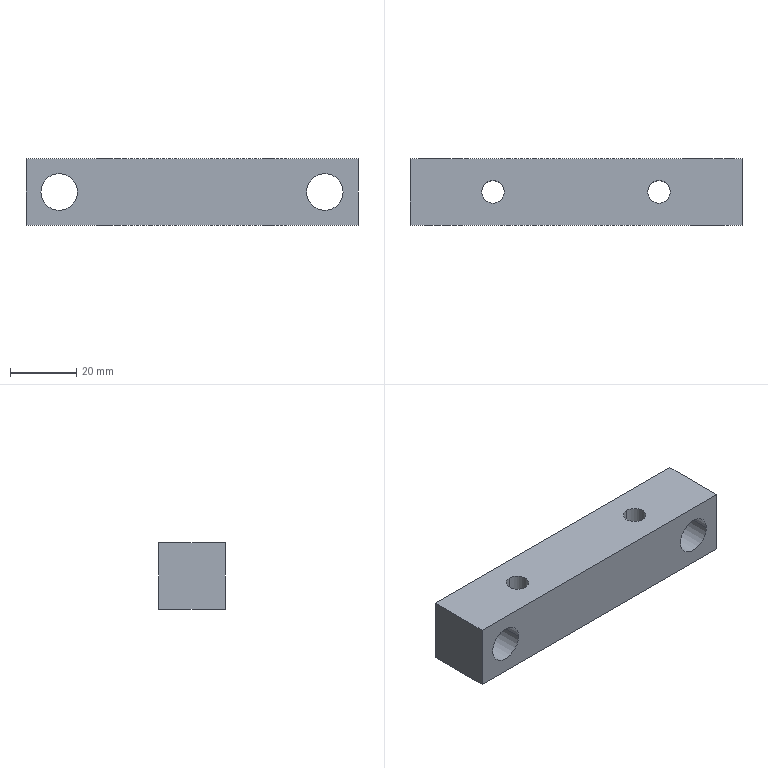Component | SolidWorks | MotorPlateFixingBlock-1 | 1 solid | 20 faces | box 100 x 20 x 20 mm | volume 33112 mm3 | cylinder 12 | plane 8 | commonest cylinder face diameters 6.8 x4 15 x4 11 x4
build123d program:
from build123d import *

# Parameters (mm, degrees)
SKETCH1_W                                        = 100
SKETCH1_H                                        = 20
EXTRUDE1_DEPTH                                   = 20
M10_HEX_SOCKET_HEAD_CAP_SCREW_CBORE1_D           = 11
M10_HEX_SOCKET_HEAD_CAP_SCREW_CBORE1_CBORE_D     = 15
M10_HEX_SOCKET_HEAD_CAP_SCREW_CBORE1_CBORE_DEPTH = 10
M8_TAPPED_HOLE1_D                                = 6.8
M8_TAPPED_HOLE1_DEPTH                            = 22.25
M8_TAPPED_HOLE1_TIP                              = 2.043


with BuildPart() as part:
    # Sketch1 → Extrude1 (new body)
    with BuildSketch(Plane.XY):
        with Locations((27.11, 12.594)):
            Rectangle(SKETCH1_W, SKETCH1_H)
    extrude(amount=EXTRUDE1_DEPTH)

    # M10 Hex Socket Head Cap Screw CBORE1 (through all)
    with Locations(Plane.XY.offset(20)):
        with Locations((67.11, 12.594), (-12.89, 12.594)):
            CounterBoreHole(M10_HEX_SOCKET_HEAD_CAP_SCREW_CBORE1_D / 2, M10_HEX_SOCKET_HEAD_CAP_SCREW_CBORE1_CBORE_D / 2, M10_HEX_SOCKET_HEAD_CAP_SCREW_CBORE1_CBORE_DEPTH)

    # M8 Tapped Hole1
    with Locations(Plane(origin=(0, 22.594, 0), x_dir=(-1, 0, 0), z_dir=(0, 1, 0))):
        with Locations((-52.11, 10), (-2.11, 10)):
            Hole(M8_TAPPED_HOLE1_D / 2, depth=M8_TAPPED_HOLE1_DEPTH)
            with Locations((0, 0, -(M8_TAPPED_HOLE1_DEPTH + M8_TAPPED_HOLE1_TIP / 2))):  # 118° drill point
                Cone(0, M8_TAPPED_HOLE1_D / 2, M8_TAPPED_HOLE1_TIP, mode=Mode.SUBTRACT)


solid = part.part

# Placed as in the assembly
solid = solid.moved(Location((-188.054, 598.983, 240.383), (-90, 0, 0)))
STEP:
#1=CARTESIAN_POINT('',(-7.321,23.842,8.574));
#2=VERTEX_POINT('',#1);
#3=CARTESIAN_POINT('',(-7.321,24.11,8.574));
#4=VERTEX_POINT('',#3);
#5=CARTESIAN_POINT('',(-7.321,23.976,8.574));
#6=DIRECTION('',(0.,0.,1.));
#7=DIRECTION('',(0.,1.,0.));
#8=AXIS2_PLACEMENT_3D('',#5,#6,#7);
#9=CIRCLE('',#8,0.1339);
#10=EDGE_CURVE('',#2,#4,#9,.T.);
#11=ORIENTED_EDGE('',*,*,#10,.F.);
#12=CARTESIAN_POINT('',(-7.321,23.842,9.362));
#13=VERTEX_POINT('',#12);
#14=CARTESIAN_POINT('',(-7.321,23.842,9.362));
#15=DIRECTION('',(0.,0.,1.));
#16=VECTOR('',#15,39.37);
#17=LINE('',#14,#16);
#18=EDGE_CURVE('',#2,#13,#17,.T.);
#19=ORIENTED_EDGE('',*,*,#18,.T.);
#20=CARTESIAN_POINT('',(-7.321,24.11,9.362));
#21=VERTEX_POINT('',#20);
#22=CARTESIAN_POINT('',(-7.321,23.976,9.362));
#23=DIRECTION('',(0.,0.,1.));
#24=DIRECTION('',(0.,1.,0.));
#25=AXIS2_PLACEMENT_3D('',#22,#23,#24);
#26=CIRCLE('',#25,0.1339);
#27=EDGE_CURVE('',#13,#21,#26,.T.);
#28=ORIENTED_EDGE('',*,*,#27,.T.);
#29=CARTESIAN_POINT('',(-7.321,24.11,9.362));
#30=DIRECTION('',(0.,0.,1.));
#31=VECTOR('',#30,39.37);
#32=LINE('',#29,#31);
#33=EDGE_CURVE('',#4,#21,#32,.T.);
#34=ORIENTED_EDGE('',*,*,#33,.F.);
#35=EDGE_LOOP('',(#11,#19,#28,#34));
#36=FACE_OUTER_BOUND('',#35,.T.);
#37=CARTESIAN_POINT('',(-7.321,23.976,9.362));
#38=DIRECTION('',(0.,0.,1.));
#39=DIRECTION('',(0.,1.,0.));
#40=AXIS2_PLACEMENT_3D('',#37,#38,#39);
#41=CYLINDRICAL_SURFACE('',#40,0.1339);
#42=ADVANCED_FACE('',(#36),#41,.F.);
#43=CARTESIAN_POINT('',(-5.352,23.842,8.574));
#44=VERTEX_POINT('',#43);
#45=CARTESIAN_POINT('',(-5.352,24.11,8.574));
#46=VERTEX_POINT('',#45);
#47=CARTESIAN_POINT('',(-5.352,23.976,8.574));
#48=DIRECTION('',(0.,0.,1.));
#49=DIRECTION('',(0.,1.,0.));
#50=AXIS2_PLACEMENT_3D('',#47,#48,#49);
#51=CIRCLE('',#50,0.1339);
#52=EDGE_CURVE('',#44,#46,#51,.T.);
#53=ORIENTED_EDGE('',*,*,#52,.F.);
#54=CARTESIAN_POINT('',(-5.352,23.842,9.362));
#55=VERTEX_POINT('',#54);
#56=CARTESIAN_POINT('',(-5.352,23.842,9.362));
#57=DIRECTION('',(0.,0.,1.));
#58=VECTOR('',#57,39.37);
#59=LINE('',#56,#58);
#60=EDGE_CURVE('',#44,#55,#59,.T.);
#61=ORIENTED_EDGE('',*,*,#60,.T.);
#62=CARTESIAN_POINT('',(-5.352,24.11,9.362));
#63=VERTEX_POINT('',#62);
#64=CARTESIAN_POINT('',(-5.352,23.976,9.362));
#65=DIRECTION('',(0.,0.,1.));
#66=DIRECTION('',(0.,1.,0.));
#67=AXIS2_PLACEMENT_3D('',#64,#65,#66);
#68=CIRCLE('',#67,0.1339);
#69=EDGE_CURVE('',#55,#63,#68,.T.);
#70=ORIENTED_EDGE('',*,*,#69,.T.);
#71=CARTESIAN_POINT('',(-5.352,24.11,9.362));
#72=DIRECTION('',(0.,0.,1.));
#73=VECTOR('',#72,39.37);
#74=LINE('',#71,#73);
#75=EDGE_CURVE('',#46,#63,#74,.T.);
#76=ORIENTED_EDGE('',*,*,#75,.F.);
#77=EDGE_LOOP('',(#53,#61,#70,#76));
#78=FACE_OUTER_BOUND('',#77,.T.);
#79=CARTESIAN_POINT('',(-5.352,23.976,9.362));
#80=DIRECTION('',(0.,0.,1.));
#81=DIRECTION('',(0.,1.,0.));
#82=AXIS2_PLACEMENT_3D('',#79,#80,#81);
#83=CYLINDRICAL_SURFACE('',#82,0.1339);
#84=ADVANCED_FACE('',(#78),#83,.F.);
#85=CARTESIAN_POINT('',(-4.466,23.976,8.968));
#86=VERTEX_POINT('',#85);
#87=CARTESIAN_POINT('',(-5.057,23.976,8.968));
#88=VERTEX_POINT('',#87);
#89=CARTESIAN_POINT('',(-4.762,23.976,8.968));
#90=DIRECTION('',(0.,1.,-0.));
#91=DIRECTION('',(-1.,0.,0.));
#92=AXIS2_PLACEMENT_3D('',#89,#90,#91);
#93=CIRCLE('',#92,0.2953);
#94=EDGE_CURVE('',#86,#88,#93,.T.);
#95=ORIENTED_EDGE('',*,*,#94,.F.);
#96=CARTESIAN_POINT('',(-4.466,24.369,8.968));
#97=VERTEX_POINT('',#96);
#98=CARTESIAN_POINT('',(-4.466,24.369,8.968));
#99=DIRECTION('',(0.,1.,-0.));
#100=VECTOR('',#99,39.37);
#101=LINE('',#98,#100);
#102=EDGE_CURVE('',#86,#97,#101,.T.);
#103=ORIENTED_EDGE('',*,*,#102,.T.);
#104=CARTESIAN_POINT('',(-5.057,24.369,8.968));
#105=VERTEX_POINT('',#104);
#106=CARTESIAN_POINT('',(-4.762,24.369,8.968));
#107=DIRECTION('',(0.,1.,-0.));
#108=DIRECTION('',(-1.,0.,0.));
#109=AXIS2_PLACEMENT_3D('',#106,#107,#108);
#110=CIRCLE('',#109,0.2953);
#111=EDGE_CURVE('',#97,#105,#110,.T.);
#112=ORIENTED_EDGE('',*,*,#111,.T.);
#113=CARTESIAN_POINT('',(-5.057,24.369,8.968));
#114=DIRECTION('',(0.,1.,-0.));
#115=VECTOR('',#114,39.37);
#116=LINE('',#113,#115);
#117=EDGE_CURVE('',#88,#105,#116,.T.);
#118=ORIENTED_EDGE('',*,*,#117,.F.);
#119=EDGE_LOOP('',(#95,#103,#112,#118));
#120=FACE_OUTER_BOUND('',#119,.T.);
#121=CARTESIAN_POINT('',(-4.762,24.369,8.968));
#122=DIRECTION('',(0.,1.,-0.));
#123=DIRECTION('',(-1.,0.,0.));
#124=AXIS2_PLACEMENT_3D('',#121,#122,#123);
#125=CYLINDRICAL_SURFACE('',#124,0.2953);
#126=ADVANCED_FACE('',(#120),#125,.F.);
#127=CARTESIAN_POINT('',(-4.545,23.582,8.968));
#128=VERTEX_POINT('',#127);
#129=CARTESIAN_POINT('',(-4.978,23.582,8.968));
#130=VERTEX_POINT('',#129);
#131=CARTESIAN_POINT('',(-4.762,23.582,8.968));
#132=DIRECTION('',(0.,1.,-0.));
#133=DIRECTION('',(-1.,0.,0.));
#134=AXIS2_PLACEMENT_3D('',#131,#132,#133);
#135=CIRCLE('',#134,0.2165);
#136=EDGE_CURVE('',#128,#130,#135,.T.);
#137=ORIENTED_EDGE('',*,*,#136,.F.);
#138=CARTESIAN_POINT('',(-4.545,23.976,8.968));
#139=VERTEX_POINT('',#138);
#140=CARTESIAN_POINT('',(-4.545,24.369,8.968));
#141=DIRECTION('',(0.,1.,-0.));
#142=VECTOR('',#141,39.37);
#143=LINE('',#140,#142);
#144=EDGE_CURVE('',#128,#139,#143,.T.);
#145=ORIENTED_EDGE('',*,*,#144,.T.);
#146=CARTESIAN_POINT('',(-4.978,23.976,8.968));
#147=VERTEX_POINT('',#146);
#148=CARTESIAN_POINT('',(-4.762,23.976,8.968));
#149=DIRECTION('',(0.,1.,-0.));
#150=DIRECTION('',(-1.,0.,0.));
#151=AXIS2_PLACEMENT_3D('',#148,#149,#150);
#152=CIRCLE('',#151,0.2165);
#153=EDGE_CURVE('',#139,#147,#152,.T.);
#154=ORIENTED_EDGE('',*,*,#153,.T.);
#155=CARTESIAN_POINT('',(-4.978,24.369,8.968));
#156=DIRECTION('',(0.,1.,-0.));
#157=VECTOR('',#156,39.37);
#158=LINE('',#155,#157);
#159=EDGE_CURVE('',#130,#147,#158,.T.);
#160=ORIENTED_EDGE('',*,*,#159,.F.);
#161=EDGE_LOOP('',(#137,#145,#154,#160));
#162=FACE_OUTER_BOUND('',#161,.T.);
#163=CARTESIAN_POINT('',(-4.762,24.369,8.968));
#164=DIRECTION('',(0.,1.,-0.));
#165=DIRECTION('',(-1.,0.,0.));
#166=AXIS2_PLACEMENT_3D('',#163,#164,#165);
#167=CYLINDRICAL_SURFACE('',#166,0.2165);
#168=ADVANCED_FACE('',(#162),#167,.F.);
#169=CARTESIAN_POINT('',(-7.616,23.976,8.968));
#170=VERTEX_POINT('',#169);
#171=CARTESIAN_POINT('',(-8.206,23.976,8.968));
#172=VERTEX_POINT('',#171);
#173=CARTESIAN_POINT('',(-7.911,23.976,8.968));
#174=DIRECTION('',(0.,1.,-0.));
#175=DIRECTION('',(-1.,0.,0.));
#176=AXIS2_PLACEMENT_3D('',#173,#174,#175);
#177=CIRCLE('',#176,0.2953);
#178=EDGE_CURVE('',#170,#172,#177,.T.);
#179=ORIENTED_EDGE('',*,*,#178,.F.);
#180=CARTESIAN_POINT('',(-7.616,24.369,8.968));
#181=VERTEX_POINT('',#180);
#182=CARTESIAN_POINT('',(-7.616,24.369,8.968));
#183=DIRECTION('',(0.,1.,-0.));
#184=VECTOR('',#183,39.37);
#185=LINE('',#182,#184);
#186=EDGE_CURVE('',#170,#181,#185,.T.);
#187=ORIENTED_EDGE('',*,*,#186,.T.);
#188=CARTESIAN_POINT('',(-8.206,24.369,8.968));
#189=VERTEX_POINT('',#188);
#190=CARTESIAN_POINT('',(-7.911,24.369,8.968));
#191=DIRECTION('',(0.,1.,-0.));
#192=DIRECTION('',(-1.,0.,0.));
#193=AXIS2_PLACEMENT_3D('',#190,#191,#192);
#194=CIRCLE('',#193,0.2953);
#195=EDGE_CURVE('',#181,#189,#194,.T.);
#196=ORIENTED_EDGE('',*,*,#195,.T.);
#197=CARTESIAN_POINT('',(-8.206,24.369,8.968));
#198=DIRECTION('',(0.,1.,-0.));
#199=VECTOR('',#198,39.37);
#200=LINE('',#197,#199);
#201=EDGE_CURVE('',#172,#189,#200,.T.);
#202=ORIENTED_EDGE('',*,*,#201,.F.);
#203=EDGE_LOOP('',(#179,#187,#196,#202));
#204=FACE_OUTER_BOUND('',#203,.T.);
#205=CARTESIAN_POINT('',(-7.911,24.369,8.968));
#206=DIRECTION('',(0.,1.,-0.));
#207=DIRECTION('',(-1.,0.,0.));
#208=AXIS2_PLACEMENT_3D('',#205,#206,#207);
#209=CYLINDRICAL_SURFACE('',#208,0.2953);
#210=ADVANCED_FACE('',(#204),#209,.F.);
#211=CARTESIAN_POINT('',(-7.695,23.582,8.968));
#212=VERTEX_POINT('',#211);
#213=CARTESIAN_POINT('',(-8.128,23.582,8.968));
#214=VERTEX_POINT('',#213);
#215=CARTESIAN_POINT('',(-7.911,23.582,8.968));
#216=DIRECTION('',(0.,1.,-0.));
#217=DIRECTION('',(-1.,0.,0.));
#218=AXIS2_PLACEMENT_3D('',#215,#216,#217);
#219=CIRCLE('',#218,0.2165);
#220=EDGE_CURVE('',#212,#214,#219,.T.);
#221=ORIENTED_EDGE('',*,*,#220,.F.);
#222=CARTESIAN_POINT('',(-7.695,23.976,8.968));
#223=VERTEX_POINT('',#222);
#224=CARTESIAN_POINT('',(-7.695,24.369,8.968));
#225=DIRECTION('',(0.,1.,-0.));
#226=VECTOR('',#225,39.37);
#227=LINE('',#224,#226);
#228=EDGE_CURVE('',#212,#223,#227,.T.);
#229=ORIENTED_EDGE('',*,*,#228,.T.);
#230=CARTESIAN_POINT('',(-8.128,23.976,8.968));
#231=VERTEX_POINT('',#230);
#232=CARTESIAN_POINT('',(-7.911,23.976,8.968));
#233=DIRECTION('',(0.,1.,-0.));
#234=DIRECTION('',(-1.,0.,0.));
#235=AXIS2_PLACEMENT_3D('',#232,#233,#234);
#236=CIRCLE('',#235,0.2165);
#237=EDGE_CURVE('',#223,#231,#236,.T.);
#238=ORIENTED_EDGE('',*,*,#237,.T.);
#239=CARTESIAN_POINT('',(-8.128,24.369,8.968));
#240=DIRECTION('',(0.,1.,-0.));
#241=VECTOR('',#240,39.37);
#242=LINE('',#239,#241);
#243=EDGE_CURVE('',#214,#231,#242,.T.);
#244=ORIENTED_EDGE('',*,*,#243,.F.);
#245=EDGE_LOOP('',(#221,#229,#238,#244));
#246=FACE_OUTER_BOUND('',#245,.T.);
#247=CARTESIAN_POINT('',(-7.911,24.369,8.968));
#248=DIRECTION('',(0.,1.,-0.));
#249=DIRECTION('',(-1.,0.,0.));
#250=AXIS2_PLACEMENT_3D('',#247,#248,#249);
#251=CYLINDRICAL_SURFACE('',#250,0.2165);
#252=ADVANCED_FACE('',(#246),#251,.F.);
#253=CARTESIAN_POINT('',(-4.368,23.582,9.362));
#254=VERTEX_POINT('',#253);
#255=CARTESIAN_POINT('',(-4.368,23.582,8.574));
#256=VERTEX_POINT('',#255);
#257=CARTESIAN_POINT('',(-4.368,23.582,9.362));
#258=DIRECTION('',(-0.,0.,-1.));
#259=VECTOR('',#258,39.37);
#260=LINE('',#257,#259);
#261=EDGE_CURVE('',#254,#256,#260,.T.);
#262=ORIENTED_EDGE('',*,*,#261,.T.);
#263=CARTESIAN_POINT('',(-4.368,24.369,8.574));
#264=VERTEX_POINT('',#263);
#265=CARTESIAN_POINT('',(-4.368,24.369,8.574));
#266=DIRECTION('',(0.,-1.,0.));
#267=VECTOR('',#266,39.37);
#268=LINE('',#265,#267);
#269=EDGE_CURVE('',#264,#256,#268,.T.);
#270=ORIENTED_EDGE('',*,*,#269,.F.);
#271=CARTESIAN_POINT('',(-4.368,24.369,9.362));
#272=VERTEX_POINT('',#271);
#273=CARTESIAN_POINT('',(-4.368,24.369,9.362));
#274=DIRECTION('',(-0.,0.,-1.));
#275=VECTOR('',#274,39.37);
#276=LINE('',#273,#275);
#277=EDGE_CURVE('',#272,#264,#276,.T.);
#278=ORIENTED_EDGE('',*,*,#277,.F.);
#279=CARTESIAN_POINT('',(-4.368,24.369,9.362));
#280=DIRECTION('',(0.,-1.,0.));
#281=VECTOR('',#280,39.37);
#282=LINE('',#279,#281);
#283=EDGE_CURVE('',#272,#254,#282,.T.);
#284=ORIENTED_EDGE('',*,*,#283,.T.);
#285=EDGE_LOOP('',(#262,#270,#278,#284));
#286=FACE_OUTER_BOUND('',#285,.T.);
#287=CARTESIAN_POINT('',(-4.368,24.369,9.362));
#288=DIRECTION('',(-1.,0.,0.));
#289=DIRECTION('',(0.,0.,1.));
#290=AXIS2_PLACEMENT_3D('',#287,#288,#289);
#291=PLANE('',#290);
#292=ADVANCED_FACE('',(#286),#291,.F.);
#293=CARTESIAN_POINT('',(-7.321,23.976,8.574));
#294=DIRECTION('',(0.,0.,1.));
#295=DIRECTION('',(0.,1.,0.));
#296=AXIS2_PLACEMENT_3D('',#293,#294,#295);
#297=CIRCLE('',#296,0.1339);
#298=EDGE_CURVE('',#4,#2,#297,.T.);
#299=ORIENTED_EDGE('',*,*,#298,.T.);
#300=ORIENTED_EDGE('',*,*,#10,.T.);
#301=EDGE_LOOP('',(#299,#300));
#302=FACE_BOUND('',#301,.T.);
#303=CARTESIAN_POINT('',(-5.352,23.976,8.574));
#304=DIRECTION('',(0.,0.,1.));
#305=DIRECTION('',(0.,1.,0.));
#306=AXIS2_PLACEMENT_3D('',#303,#304,#305);
#307=CIRCLE('',#306,0.1339);
#308=EDGE_CURVE('',#46,#44,#307,.T.);
#309=ORIENTED_EDGE('',*,*,#308,.T.);
#310=ORIENTED_EDGE('',*,*,#52,.T.);
#311=EDGE_LOOP('',(#309,#310));
#312=FACE_BOUND('',#311,.T.);
#313=CARTESIAN_POINT('',(-8.305,23.582,8.574));
#314=VERTEX_POINT('',#313);
#315=CARTESIAN_POINT('',(-4.368,23.582,8.574));
#316=DIRECTION('',(-1.,0.,0.));
#317=VECTOR('',#316,39.37);
#318=LINE('',#315,#317);
#319=EDGE_CURVE('',#256,#314,#318,.T.);
#320=ORIENTED_EDGE('',*,*,#319,.T.);
#321=CARTESIAN_POINT('',(-8.305,24.369,8.574));
#322=VERTEX_POINT('',#321);
#323=CARTESIAN_POINT('',(-8.305,24.369,8.574));
#324=DIRECTION('',(0.,-1.,0.));
#325=VECTOR('',#324,39.37);
#326=LINE('',#323,#325);
#327=EDGE_CURVE('',#322,#314,#326,.T.);
#328=ORIENTED_EDGE('',*,*,#327,.F.);
#329=CARTESIAN_POINT('',(-4.368,24.369,8.574));
#330=DIRECTION('',(-1.,0.,0.));
#331=VECTOR('',#330,39.37);
#332=LINE('',#329,#331);
#333=EDGE_CURVE('',#264,#322,#332,.T.);
#334=ORIENTED_EDGE('',*,*,#333,.F.);
#335=ORIENTED_EDGE('',*,*,#269,.T.);
#336=EDGE_LOOP('',(#320,#328,#334,#335));
#337=FACE_OUTER_BOUND('',#336,.T.);
#338=CARTESIAN_POINT('',(-4.368,24.369,8.574));
#339=DIRECTION('',(0.,0.,1.));
#340=DIRECTION('',(0.,1.,-0.));
#341=AXIS2_PLACEMENT_3D('',#338,#339,#340);
#342=PLANE('',#341);
#343=ADVANCED_FACE('',(#302,#312,#337),#342,.F.);
#344=CARTESIAN_POINT('',(-8.305,23.582,9.362));
#345=VERTEX_POINT('',#344);
#346=CARTESIAN_POINT('',(-8.305,23.582,9.362));
#347=DIRECTION('',(0.,0.,1.));
#348=VECTOR('',#347,39.37);
#349=LINE('',#346,#348);
#350=EDGE_CURVE('',#314,#345,#349,.T.);
#351=ORIENTED_EDGE('',*,*,#350,.T.);
#352=CARTESIAN_POINT('',(-8.305,24.369,9.362));
#353=VERTEX_POINT('',#352);
#354=CARTESIAN_POINT('',(-8.305,24.369,9.362));
#355=DIRECTION('',(0.,-1.,0.));
#356=VECTOR('',#355,39.37);
#357=LINE('',#354,#356);
#358=EDGE_CURVE('',#353,#345,#357,.T.);
#359=ORIENTED_EDGE('',*,*,#358,.F.);
#360=CARTESIAN_POINT('',(-8.305,24.369,9.362));
#361=DIRECTION('',(0.,0.,1.));
#362=VECTOR('',#361,39.37);
#363=LINE('',#360,#362);
#364=EDGE_CURVE('',#322,#353,#363,.T.);
#365=ORIENTED_EDGE('',*,*,#364,.F.);
#366=ORIENTED_EDGE('',*,*,#327,.T.);
#367=EDGE_LOOP('',(#351,#359,#365,#366));
#368=FACE_OUTER_BOUND('',#367,.T.);
#369=CARTESIAN_POINT('',(-8.305,24.369,9.362));
#370=DIRECTION('',(1.,0.,0.));
#371=DIRECTION('',(0.,1.,-0.));
#372=AXIS2_PLACEMENT_3D('',#369,#370,#371);
#373=PLANE('',#372);
#374=ADVANCED_FACE('',(#368),#373,.F.);
#375=CARTESIAN_POINT('',(-7.321,23.976,9.362));
#376=DIRECTION('',(0.,0.,1.));
#377=DIRECTION('',(0.,1.,0.));
#378=AXIS2_PLACEMENT_3D('',#375,#376,#377);
#379=CIRCLE('',#378,0.1339);
#380=EDGE_CURVE('',#21,#13,#379,.T.);
#381=ORIENTED_EDGE('',*,*,#380,.F.);
#382=ORIENTED_EDGE('',*,*,#27,.F.);
#383=EDGE_LOOP('',(#381,#382));
#384=FACE_BOUND('',#383,.T.);
#385=CARTESIAN_POINT('',(-5.352,23.976,9.362));
#386=DIRECTION('',(0.,0.,1.));
#387=DIRECTION('',(0.,1.,0.));
#388=AXIS2_PLACEMENT_3D('',#385,#386,#387);
#389=CIRCLE('',#388,0.1339);
#390=EDGE_CURVE('',#63,#55,#389,.T.);
#391=ORIENTED_EDGE('',*,*,#390,.F.);
#392=ORIENTED_EDGE('',*,*,#69,.F.);
#393=EDGE_LOOP('',(#391,#392));
#394=FACE_BOUND('',#393,.T.);
#395=CARTESIAN_POINT('',(-4.368,23.582,9.362));
#396=DIRECTION('',(1.,0.,0.));
#397=VECTOR('',#396,39.37);
#398=LINE('',#395,#397);
#399=EDGE_CURVE('',#345,#254,#398,.T.);
#400=ORIENTED_EDGE('',*,*,#399,.T.);
#401=ORIENTED_EDGE('',*,*,#283,.F.);
#402=CARTESIAN_POINT('',(-4.368,24.369,9.362));
#403=DIRECTION('',(1.,0.,0.));
#404=VECTOR('',#403,39.37);
#405=LINE('',#402,#404);
#406=EDGE_CURVE('',#353,#272,#405,.T.);
#407=ORIENTED_EDGE('',*,*,#406,.F.);
#408=ORIENTED_EDGE('',*,*,#358,.T.);
#409=EDGE_LOOP('',(#400,#401,#407,#408));
#410=FACE_OUTER_BOUND('',#409,.T.);
#411=CARTESIAN_POINT('',(-4.368,24.369,9.362));
#412=DIRECTION('',(0.,-0.,-1.));
#413=DIRECTION('',(0.,-1.,0.));
#414=AXIS2_PLACEMENT_3D('',#411,#412,#413);
#415=PLANE('',#414);
#416=ADVANCED_FACE('',(#384,#394,#410),#415,.F.);
#417=CARTESIAN_POINT('',(-4.762,24.369,8.968));
#418=DIRECTION('',(0.,1.,-0.));
#419=DIRECTION('',(-1.,0.,0.));
#420=AXIS2_PLACEMENT_3D('',#417,#418,#419);
#421=CIRCLE('',#420,0.2953);
#422=EDGE_CURVE('',#105,#97,#421,.T.);
#423=ORIENTED_EDGE('',*,*,#422,.F.);
#424=ORIENTED_EDGE('',*,*,#111,.F.);
#425=EDGE_LOOP('',(#423,#424));
#426=FACE_BOUND('',#425,.T.);
#427=CARTESIAN_POINT('',(-7.911,24.369,8.968));
#428=DIRECTION('',(0.,1.,-0.));
#429=DIRECTION('',(-1.,0.,0.));
#430=AXIS2_PLACEMENT_3D('',#427,#428,#429);
#431=CIRCLE('',#430,0.2953);
#432=EDGE_CURVE('',#189,#181,#431,.T.);
#433=ORIENTED_EDGE('',*,*,#432,.F.);
#434=ORIENTED_EDGE('',*,*,#195,.F.);
#435=EDGE_LOOP('',(#433,#434));
#436=FACE_BOUND('',#435,.T.);
#437=ORIENTED_EDGE('',*,*,#277,.T.);
#438=ORIENTED_EDGE('',*,*,#333,.T.);
#439=ORIENTED_EDGE('',*,*,#364,.T.);
#440=ORIENTED_EDGE('',*,*,#406,.T.);
#441=EDGE_LOOP('',(#437,#438,#439,#440));
#442=FACE_OUTER_BOUND('',#441,.T.);
#443=CARTESIAN_POINT('',(-4.368,24.369,8.574));
#444=DIRECTION('',(0.,1.,-0.));
#445=DIRECTION('',(-1.,0.,0.));
#446=AXIS2_PLACEMENT_3D('',#443,#444,#445);
#447=PLANE('',#446);
#448=ADVANCED_FACE('',(#426,#436,#442),#447,.T.);
#449=CARTESIAN_POINT('',(-4.762,23.582,8.968));
#450=DIRECTION('',(0.,1.,-0.));
#451=DIRECTION('',(-1.,0.,0.));
#452=AXIS2_PLACEMENT_3D('',#449,#450,#451);
#453=CIRCLE('',#452,0.2165);
#454=EDGE_CURVE('',#130,#128,#453,.T.);
#455=ORIENTED_EDGE('',*,*,#454,.T.);
#456=ORIENTED_EDGE('',*,*,#136,.T.);
#457=EDGE_LOOP('',(#455,#456));
#458=FACE_BOUND('',#457,.T.);
#459=CARTESIAN_POINT('',(-7.911,23.582,8.968));
#460=DIRECTION('',(0.,1.,-0.));
#461=DIRECTION('',(-1.,0.,0.));
#462=AXIS2_PLACEMENT_3D('',#459,#460,#461);
#463=CIRCLE('',#462,0.2165);
#464=EDGE_CURVE('',#214,#212,#463,.T.);
#465=ORIENTED_EDGE('',*,*,#464,.T.);
#466=ORIENTED_EDGE('',*,*,#220,.T.);
#467=EDGE_LOOP('',(#465,#466));
#468=FACE_BOUND('',#467,.T.);
#469=ORIENTED_EDGE('',*,*,#261,.F.);
#470=ORIENTED_EDGE('',*,*,#399,.F.);
#471=ORIENTED_EDGE('',*,*,#350,.F.);
#472=ORIENTED_EDGE('',*,*,#319,.F.);
#473=EDGE_LOOP('',(#469,#470,#471,#472));
#474=FACE_OUTER_BOUND('',#473,.T.);
#475=CARTESIAN_POINT('',(-4.368,23.582,8.574));
#476=DIRECTION('',(0.,1.,-0.));
#477=DIRECTION('',(-1.,0.,0.));
#478=AXIS2_PLACEMENT_3D('',#475,#476,#477);
#479=PLANE('',#478);
#480=ADVANCED_FACE('',(#458,#468,#474),#479,.F.);
#481=ORIENTED_EDGE('',*,*,#228,.F.);
#482=ORIENTED_EDGE('',*,*,#464,.F.);
#483=ORIENTED_EDGE('',*,*,#243,.T.);
#484=CARTESIAN_POINT('',(-7.911,23.976,8.968));
#485=DIRECTION('',(0.,1.,-0.));
#486=DIRECTION('',(-1.,0.,0.));
#487=AXIS2_PLACEMENT_3D('',#484,#485,#486);
#488=CIRCLE('',#487,0.2165);
#489=EDGE_CURVE('',#231,#223,#488,.T.);
#490=ORIENTED_EDGE('',*,*,#489,.T.);
#491=EDGE_LOOP('',(#481,#482,#483,#490));
#492=FACE_OUTER_BOUND('',#491,.T.);
#493=CARTESIAN_POINT('',(-7.911,24.369,8.968));
#494=DIRECTION('',(0.,1.,-0.));
#495=DIRECTION('',(-1.,0.,0.));
#496=AXIS2_PLACEMENT_3D('',#493,#494,#495);
#497=CYLINDRICAL_SURFACE('',#496,0.2165);
#498=ADVANCED_FACE('',(#492),#497,.F.);
#499=ORIENTED_EDGE('',*,*,#489,.F.);
#500=ORIENTED_EDGE('',*,*,#237,.F.);
#501=EDGE_LOOP('',(#499,#500));
#502=FACE_BOUND('',#501,.T.);
#503=CARTESIAN_POINT('',(-7.911,23.976,8.968));
#504=DIRECTION('',(0.,1.,-0.));
#505=DIRECTION('',(-1.,0.,0.));
#506=AXIS2_PLACEMENT_3D('',#503,#504,#505);
#507=CIRCLE('',#506,0.2953);
#508=EDGE_CURVE('',#172,#170,#507,.T.);
#509=ORIENTED_EDGE('',*,*,#508,.T.);
#510=ORIENTED_EDGE('',*,*,#178,.T.);
#511=EDGE_LOOP('',(#509,#510));
#512=FACE_OUTER_BOUND('',#511,.T.);
#513=CARTESIAN_POINT('',(-8.128,23.976,8.968));
#514=DIRECTION('',(0.,-1.,0.));
#515=DIRECTION('',(1.,0.,0.));
#516=AXIS2_PLACEMENT_3D('',#513,#514,#515);
#517=PLANE('',#516);
#518=ADVANCED_FACE('',(#502,#512),#517,.F.);
#519=ORIENTED_EDGE('',*,*,#186,.F.);
#520=ORIENTED_EDGE('',*,*,#508,.F.);
#521=ORIENTED_EDGE('',*,*,#201,.T.);
#522=ORIENTED_EDGE('',*,*,#432,.T.);
#523=EDGE_LOOP('',(#519,#520,#521,#522));
#524=FACE_OUTER_BOUND('',#523,.T.);
#525=CARTESIAN_POINT('',(-7.911,24.369,8.968));
#526=DIRECTION('',(0.,1.,-0.));
#527=DIRECTION('',(-1.,0.,0.));
#528=AXIS2_PLACEMENT_3D('',#525,#526,#527);
#529=CYLINDRICAL_SURFACE('',#528,0.2953);
#530=ADVANCED_FACE('',(#524),#529,.F.);
#531=ORIENTED_EDGE('',*,*,#144,.F.);
#532=ORIENTED_EDGE('',*,*,#454,.F.);
#533=ORIENTED_EDGE('',*,*,#159,.T.);
#534=CARTESIAN_POINT('',(-4.762,23.976,8.968));
#535=DIRECTION('',(0.,1.,-0.));
#536=DIRECTION('',(-1.,0.,0.));
#537=AXIS2_PLACEMENT_3D('',#534,#535,#536);
#538=CIRCLE('',#537,0.2165);
#539=EDGE_CURVE('',#147,#139,#538,.T.);
#540=ORIENTED_EDGE('',*,*,#539,.T.);
#541=EDGE_LOOP('',(#531,#532,#533,#540));
#542=FACE_OUTER_BOUND('',#541,.T.);
#543=CARTESIAN_POINT('',(-4.762,24.369,8.968));
#544=DIRECTION('',(0.,1.,-0.));
#545=DIRECTION('',(-1.,0.,0.));
#546=AXIS2_PLACEMENT_3D('',#543,#544,#545);
#547=CYLINDRICAL_SURFACE('',#546,0.2165);
#548=ADVANCED_FACE('',(#542),#547,.F.);
#549=ORIENTED_EDGE('',*,*,#539,.F.);
#550=ORIENTED_EDGE('',*,*,#153,.F.);
#551=EDGE_LOOP('',(#549,#550));
#552=FACE_BOUND('',#551,.T.);
#553=CARTESIAN_POINT('',(-4.762,23.976,8.968));
#554=DIRECTION('',(0.,1.,-0.));
#555=DIRECTION('',(-1.,0.,0.));
#556=AXIS2_PLACEMENT_3D('',#553,#554,#555);
#557=CIRCLE('',#556,0.2953);
#558=EDGE_CURVE('',#88,#86,#557,.T.);
#559=ORIENTED_EDGE('',*,*,#558,.T.);
#560=ORIENTED_EDGE('',*,*,#94,.T.);
#561=EDGE_LOOP('',(#559,#560));
#562=FACE_OUTER_BOUND('',#561,.T.);
#563=CARTESIAN_POINT('',(-4.978,23.976,8.968));
#564=DIRECTION('',(0.,-1.,0.));
#565=DIRECTION('',(1.,0.,0.));
#566=AXIS2_PLACEMENT_3D('',#563,#564,#565);
#567=PLANE('',#566);
#568=ADVANCED_FACE('',(#552,#562),#567,.F.);
#569=ORIENTED_EDGE('',*,*,#102,.F.);
#570=ORIENTED_EDGE('',*,*,#558,.F.);
#571=ORIENTED_EDGE('',*,*,#117,.T.);
#572=ORIENTED_EDGE('',*,*,#422,.T.);
#573=EDGE_LOOP('',(#569,#570,#571,#572));
#574=FACE_OUTER_BOUND('',#573,.T.);
#575=CARTESIAN_POINT('',(-4.762,24.369,8.968));
#576=DIRECTION('',(0.,1.,-0.));
#577=DIRECTION('',(-1.,0.,0.));
#578=AXIS2_PLACEMENT_3D('',#575,#576,#577);
#579=CYLINDRICAL_SURFACE('',#578,0.2953);
#580=ADVANCED_FACE('',(#574),#579,.F.);
#581=ORIENTED_EDGE('',*,*,#60,.F.);
#582=ORIENTED_EDGE('',*,*,#308,.F.);
#583=ORIENTED_EDGE('',*,*,#75,.T.);
#584=ORIENTED_EDGE('',*,*,#390,.T.);
#585=EDGE_LOOP('',(#581,#582,#583,#584));
#586=FACE_OUTER_BOUND('',#585,.T.);
#587=CARTESIAN_POINT('',(-5.352,23.976,9.362));
#588=DIRECTION('',(0.,0.,1.));
#589=DIRECTION('',(0.,1.,0.));
#590=AXIS2_PLACEMENT_3D('',#587,#588,#589);
#591=CYLINDRICAL_SURFACE('',#590,0.1339);
#592=ADVANCED_FACE('',(#586),#591,.F.);
#593=ORIENTED_EDGE('',*,*,#18,.F.);
#594=ORIENTED_EDGE('',*,*,#298,.F.);
#595=ORIENTED_EDGE('',*,*,#33,.T.);
#596=ORIENTED_EDGE('',*,*,#380,.T.);
#597=EDGE_LOOP('',(#593,#594,#595,#596));
#598=FACE_OUTER_BOUND('',#597,.T.);
#599=CARTESIAN_POINT('',(-7.321,23.976,9.362));
#600=DIRECTION('',(0.,0.,1.));
#601=DIRECTION('',(0.,1.,0.));
#602=AXIS2_PLACEMENT_3D('',#599,#600,#601);
#603=CYLINDRICAL_SURFACE('',#602,0.1339);
#604=ADVANCED_FACE('',(#598),#603,.F.);
#605=CLOSED_SHELL('',(#42,#84,#126,#168,#210,#252,#292,#343,#374,#416,#448,#480,#498,#518,#530,#548,#568,#580,#592,#604));
#606=MANIFOLD_SOLID_BREP('',#605);
#607=CARTESIAN_POINT('',(0.,0.,0.));
#608=DIRECTION('',(0.,0.,1.));
#609=DIRECTION('',(1.,0.,0.));
#610=AXIS2_PLACEMENT_3D('',#607,#608,#609);
#611=(LENGTH_UNIT()NAMED_UNIT(*)SI_UNIT($,.METRE.));
#612=LENGTH_MEASURE_WITH_UNIT(LENGTH_MEASURE(0.0254),#611);
#613=DIMENSIONAL_EXPONENTS(1.,0.,0.,0.,0.,0.,0.);
#614=(CONVERSION_BASED_UNIT('',#612)LENGTH_UNIT()NAMED_UNIT(#613));
#615=UNCERTAINTY_MEASURE_WITH_UNIT(LENGTH_MEASURE(0.00001),#614,'','');
#616=(NAMED_UNIT(*)PLANE_ANGLE_UNIT()SI_UNIT($,.RADIAN.));
#617=(NAMED_UNIT(*)SI_UNIT($,.STERADIAN.)SOLID_ANGLE_UNIT());
#618=(GEOMETRIC_REPRESENTATION_CONTEXT(3)GLOBAL_UNCERTAINTY_ASSIGNED_CONTEXT((#615))GLOBAL_UNIT_ASSIGNED_CONTEXT((#614,#616,#617))REPRESENTATION_CONTEXT('',''));
#619=ADVANCED_BREP_SHAPE_REPRESENTATION('',(#606,#610),#618);
#620=COLOUR_RGB('',0.7922,0.8196,0.9333);
#621=FILL_AREA_STYLE_COLOUR('',#620);
#622=FILL_AREA_STYLE('',(#621));
#623=SURFACE_STYLE_FILL_AREA(#622);
#624=SURFACE_SIDE_STYLE('',(#623));
#625=SURFACE_STYLE_USAGE(.BOTH.,#624);
#626=PRESENTATION_STYLE_ASSIGNMENT((#625));
#627=STYLED_ITEM('',(#626),#606);
#628=PRESENTATION_LAYER_ASSIGNMENT('','',(#627));
#629=(LENGTH_UNIT()NAMED_UNIT(*)SI_UNIT($,.METRE.));
#630=LENGTH_MEASURE_WITH_UNIT(LENGTH_MEASURE(0.0254),#629);
#631=DIMENSIONAL_EXPONENTS(1.,0.,0.,0.,0.,0.,0.);
#632=(CONVERSION_BASED_UNIT('',#630)LENGTH_UNIT()NAMED_UNIT(#631));
#633=UNCERTAINTY_MEASURE_WITH_UNIT(LENGTH_MEASURE(0.00001),#632,'','');
#634=(NAMED_UNIT(*)PLANE_ANGLE_UNIT()SI_UNIT($,.RADIAN.));
#635=(NAMED_UNIT(*)SI_UNIT($,.STERADIAN.)SOLID_ANGLE_UNIT());
#636=(GEOMETRIC_REPRESENTATION_CONTEXT(3)GLOBAL_UNCERTAINTY_ASSIGNED_CONTEXT((#633))GLOBAL_UNIT_ASSIGNED_CONTEXT((#632,#634,#635))REPRESENTATION_CONTEXT('',''));
#637=MECHANICAL_DESIGN_GEOMETRIC_PRESENTATION_REPRESENTATION('',(#627),#636);